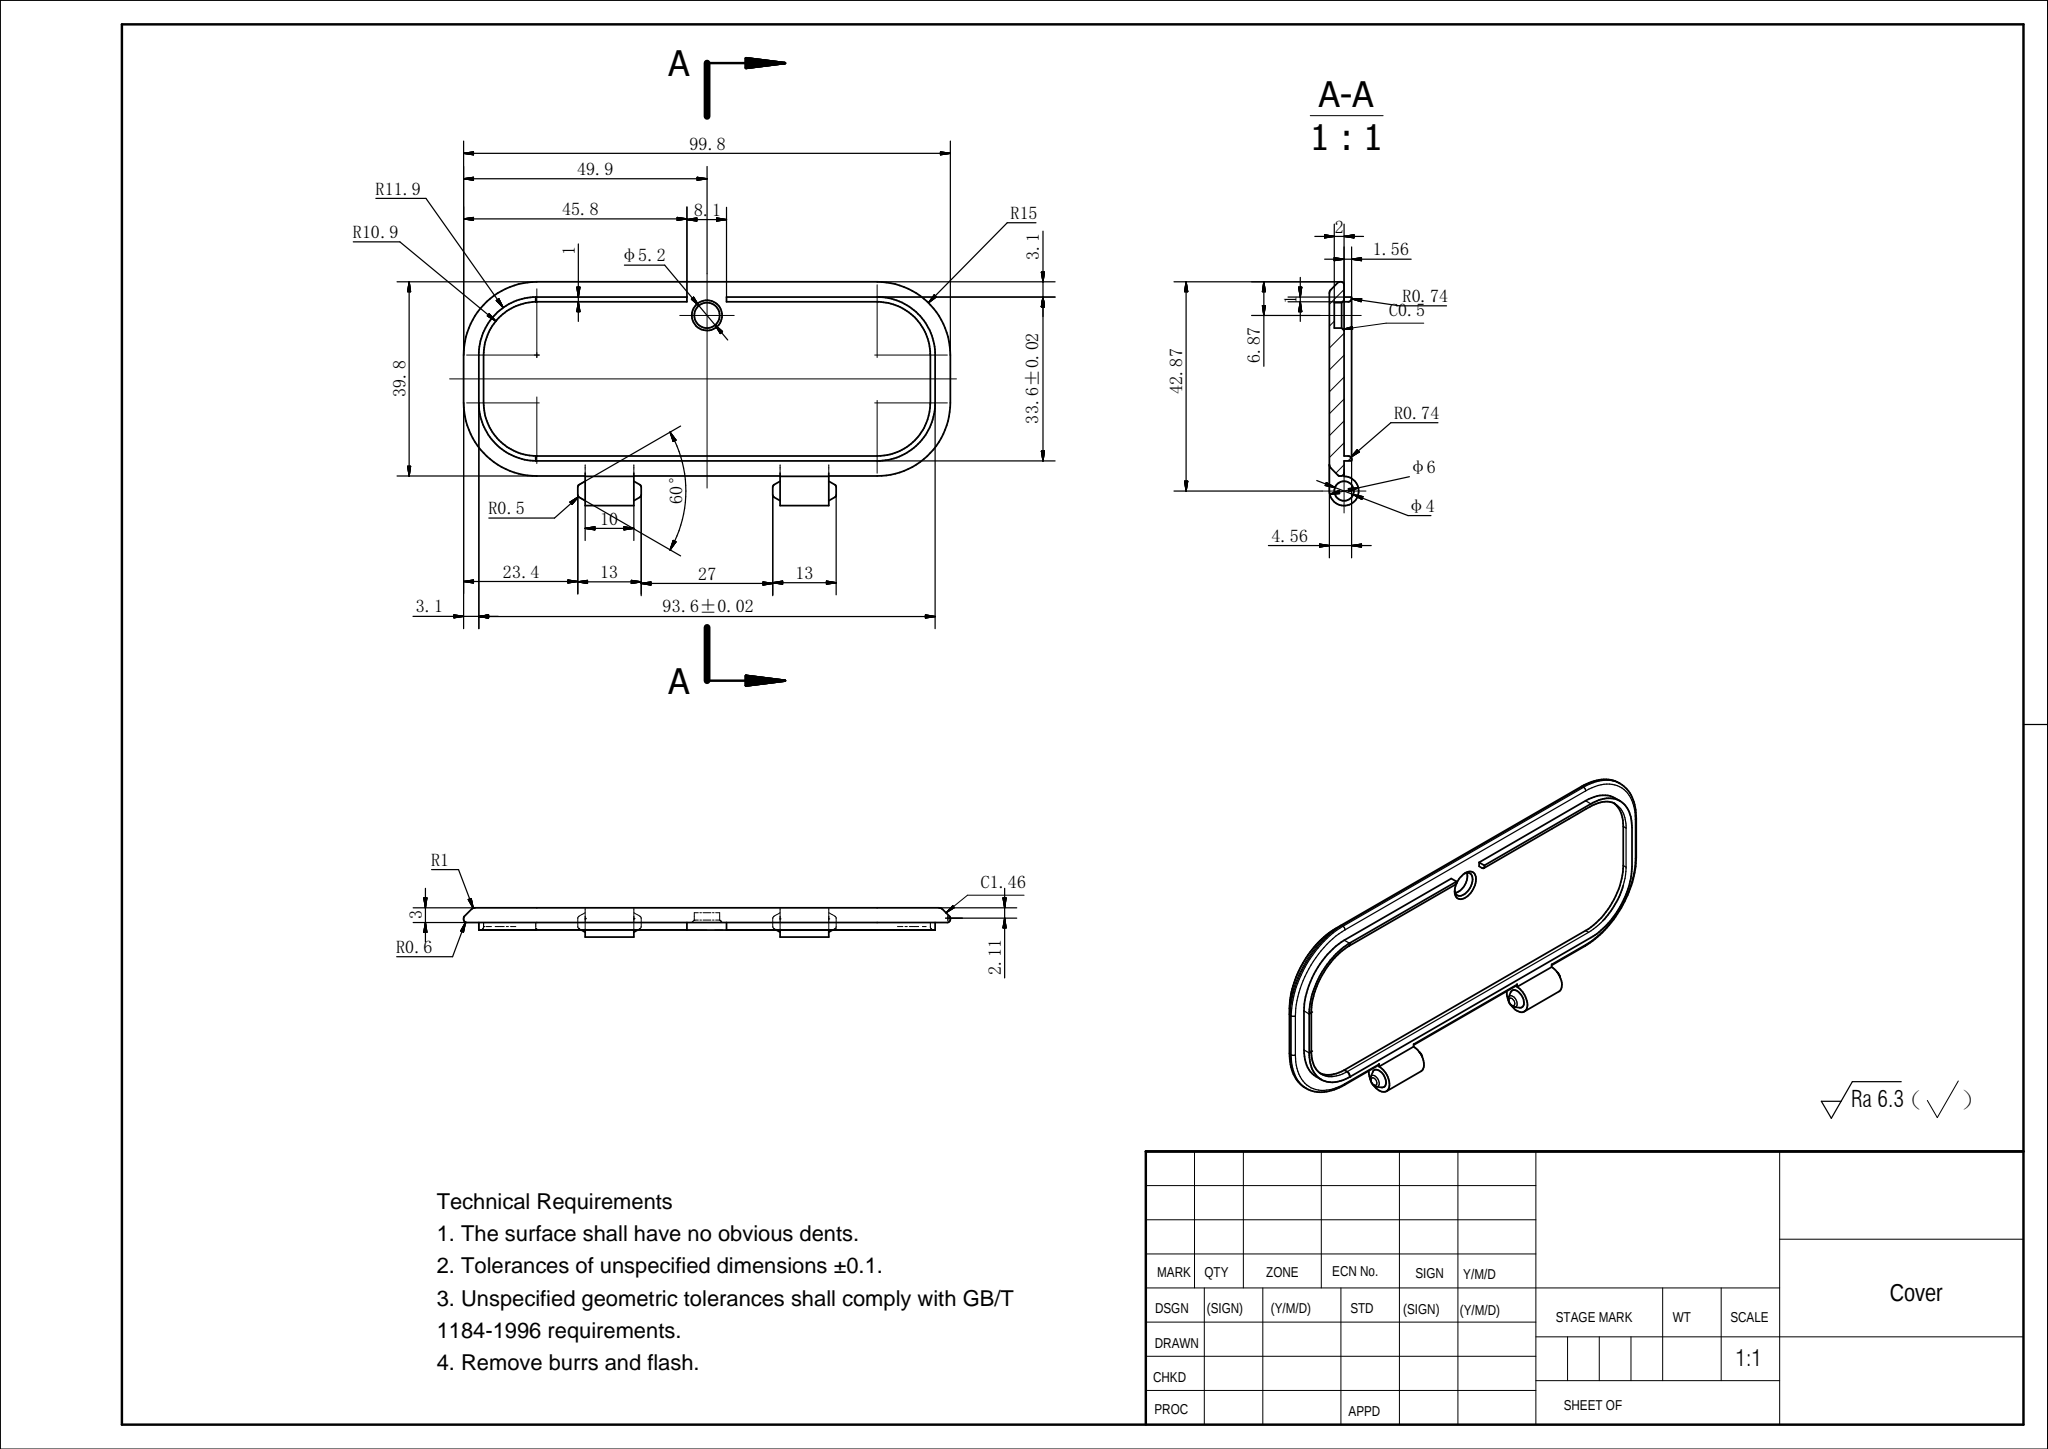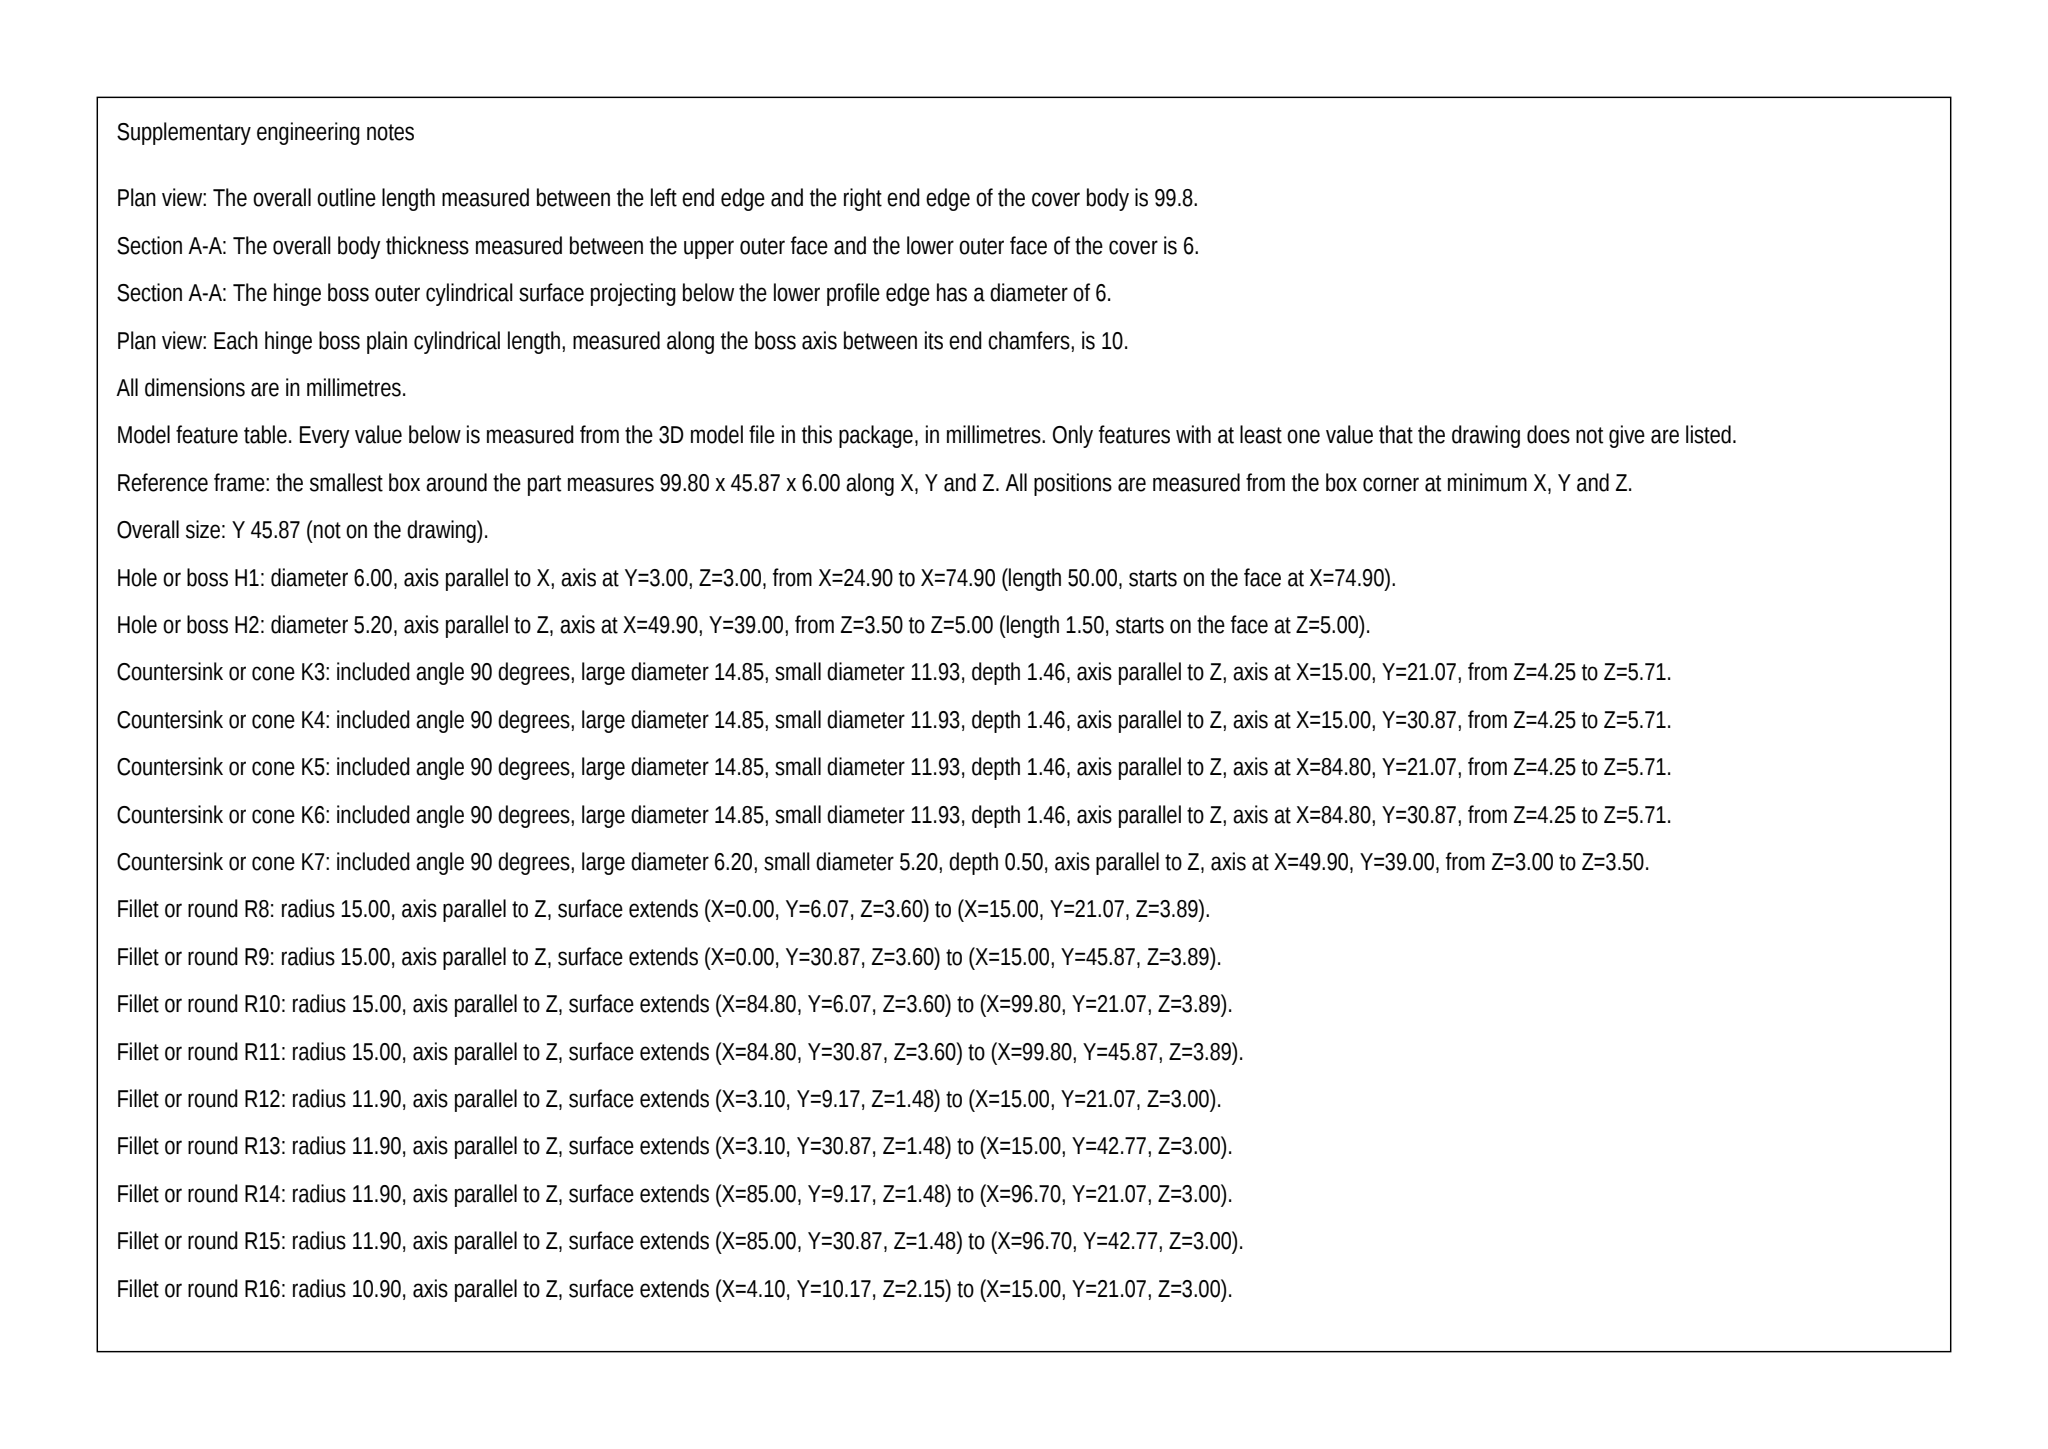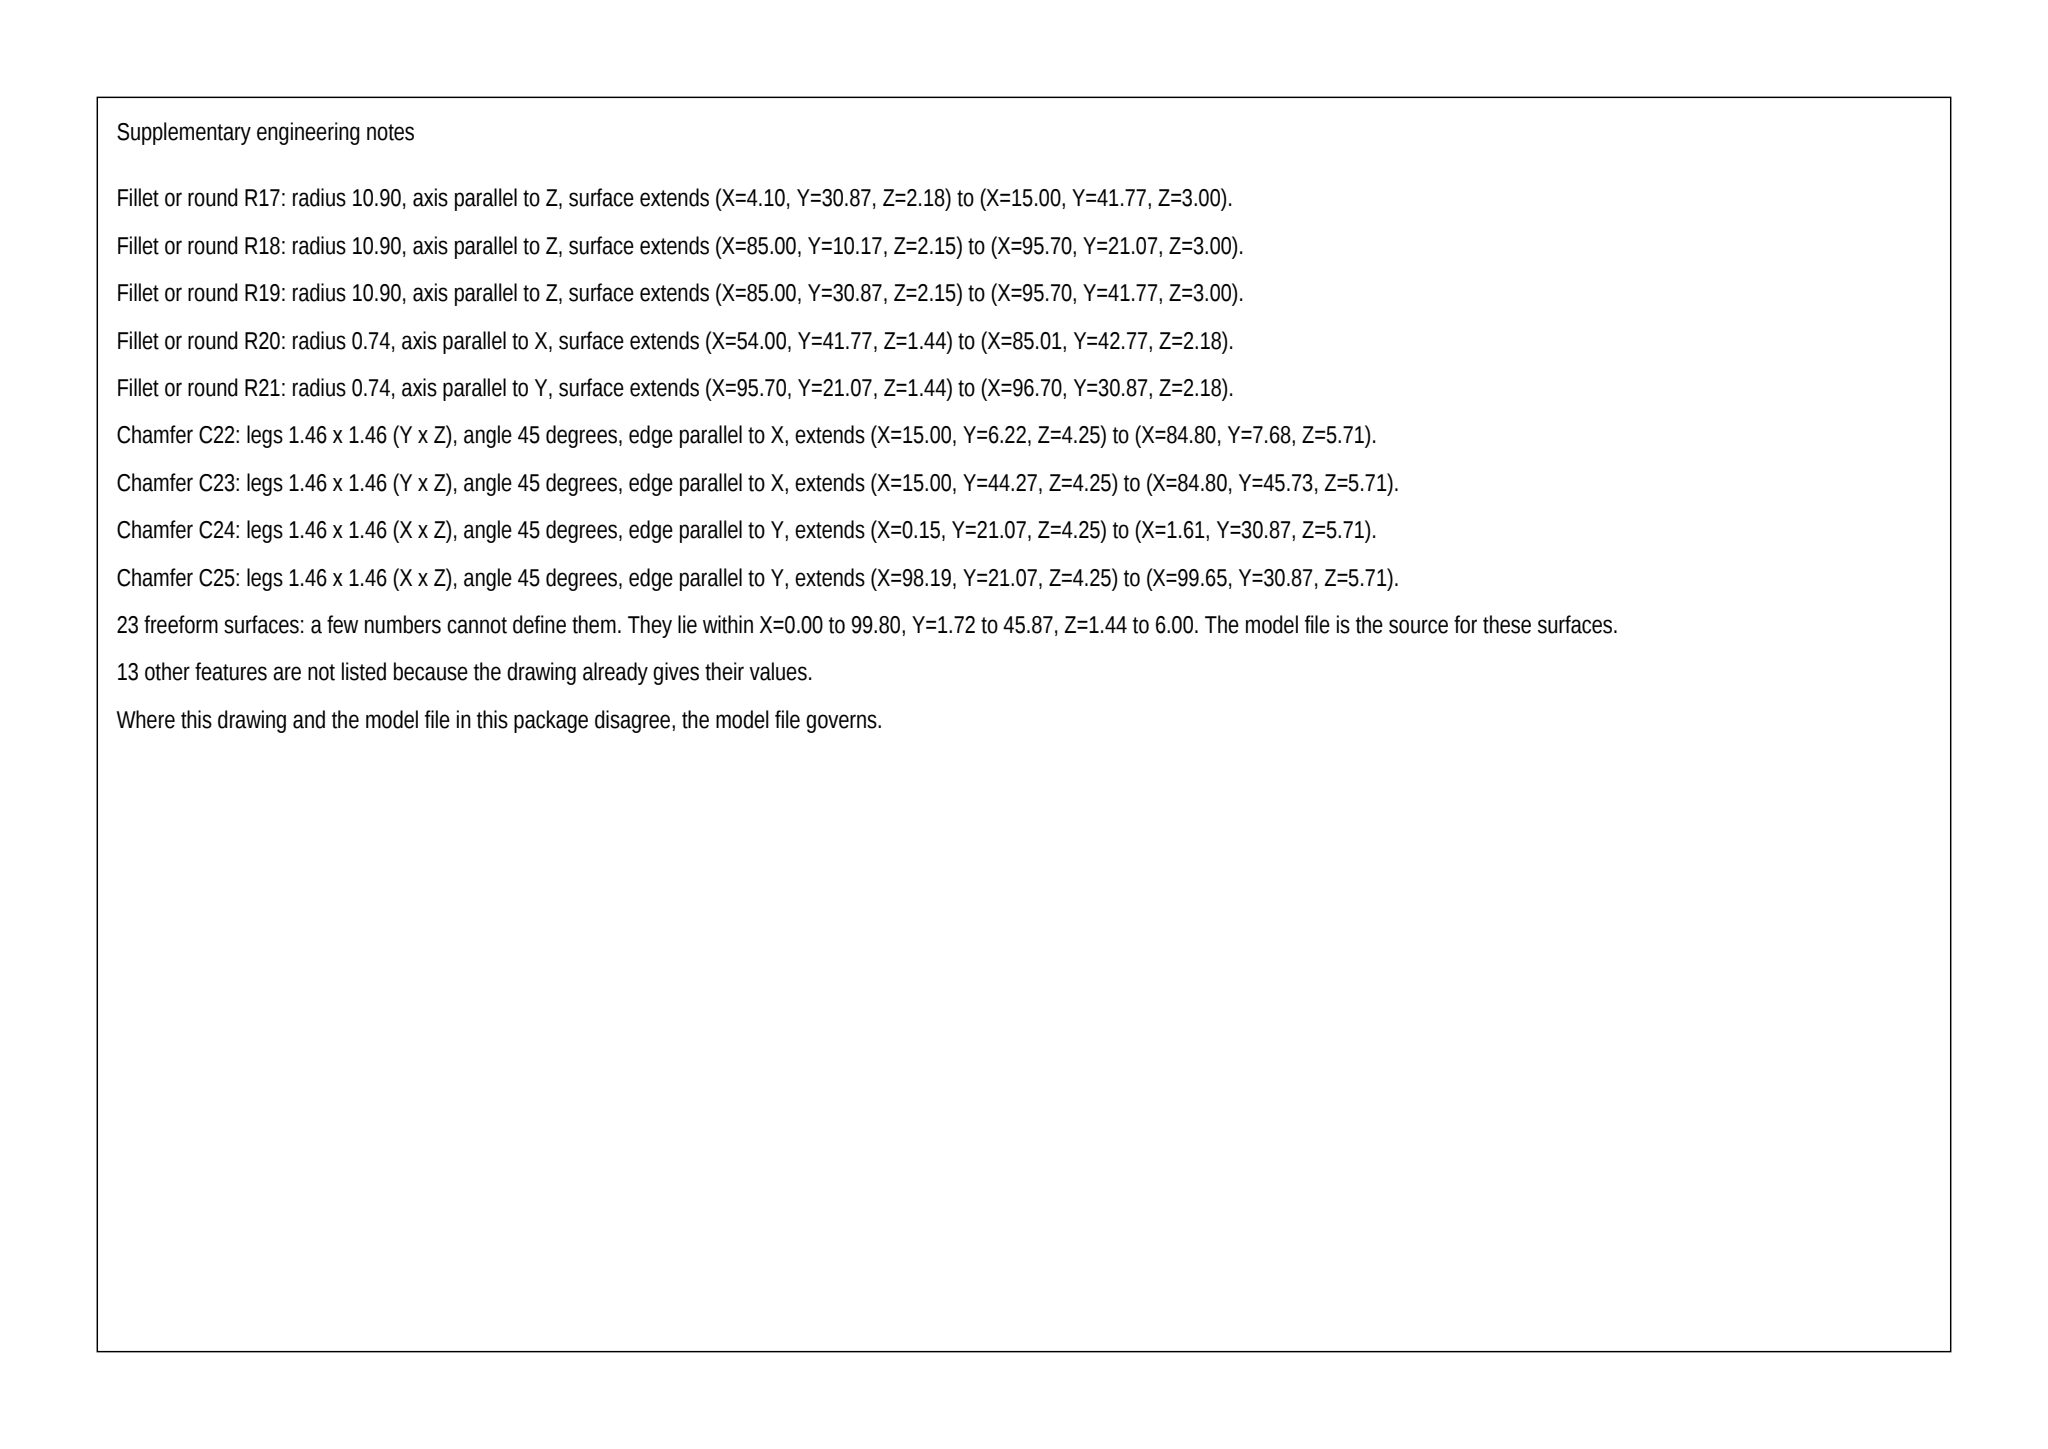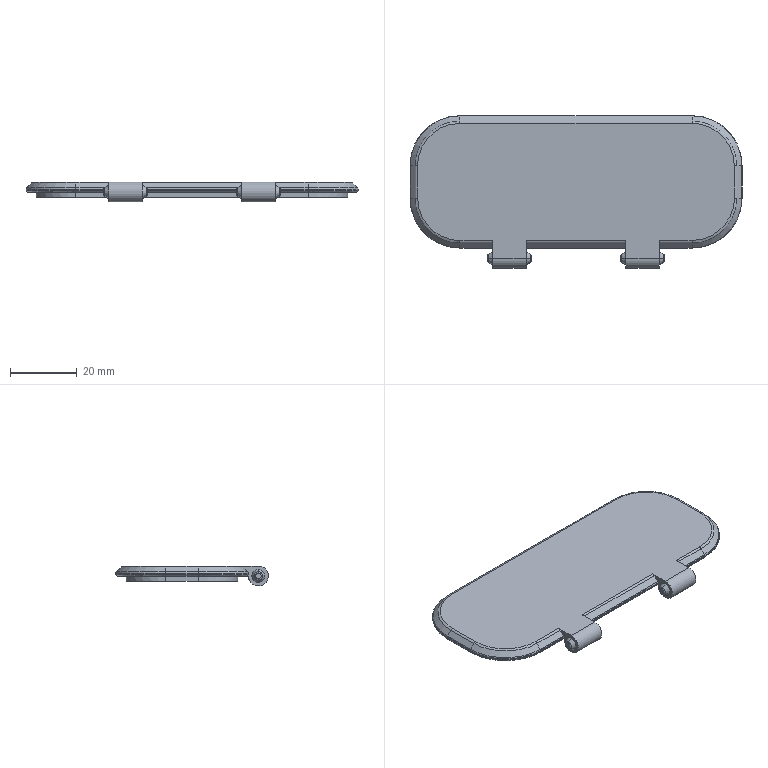Part | SolidWorks | mm | 1 solid | 113 faces | box 99.8 x 45.87 x 6 mm | volume 11832 mm3 | cylinder 41 | plane 35 | spline 23 | cone 14 | commonest cylinder face diameters 21.8 x6 23.8 x6 1.2 x6 1 x6 2 x6 30 x4 6 x3 5.2 x2